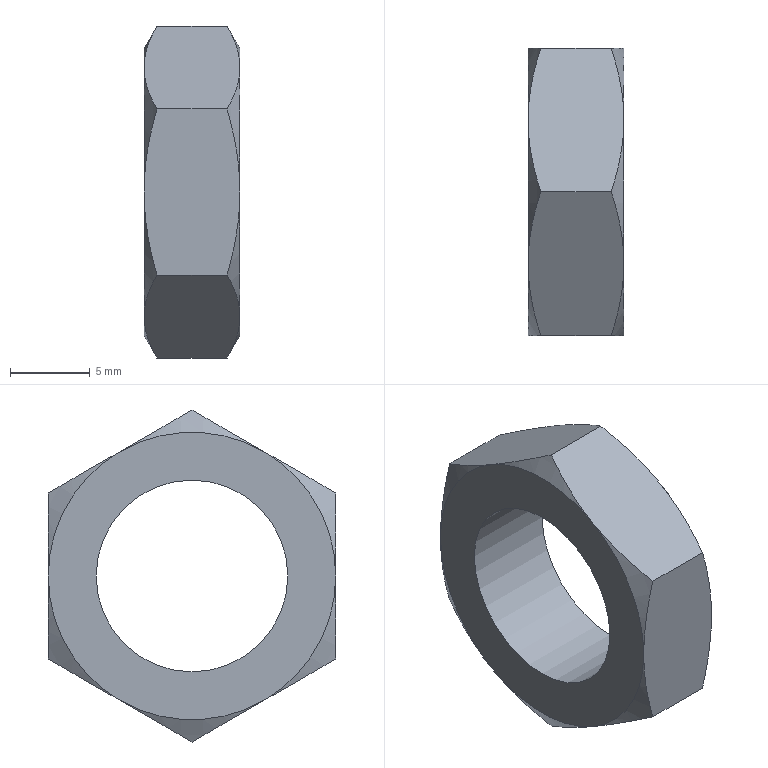Component | NX | GB-T6172_1-2000_M12X1_75 | 1 solid | 21 faces | volume 992 mm3 | cone 12 | plane 8 | cylinder 1 | commonest cylinder face diameters 12 x1